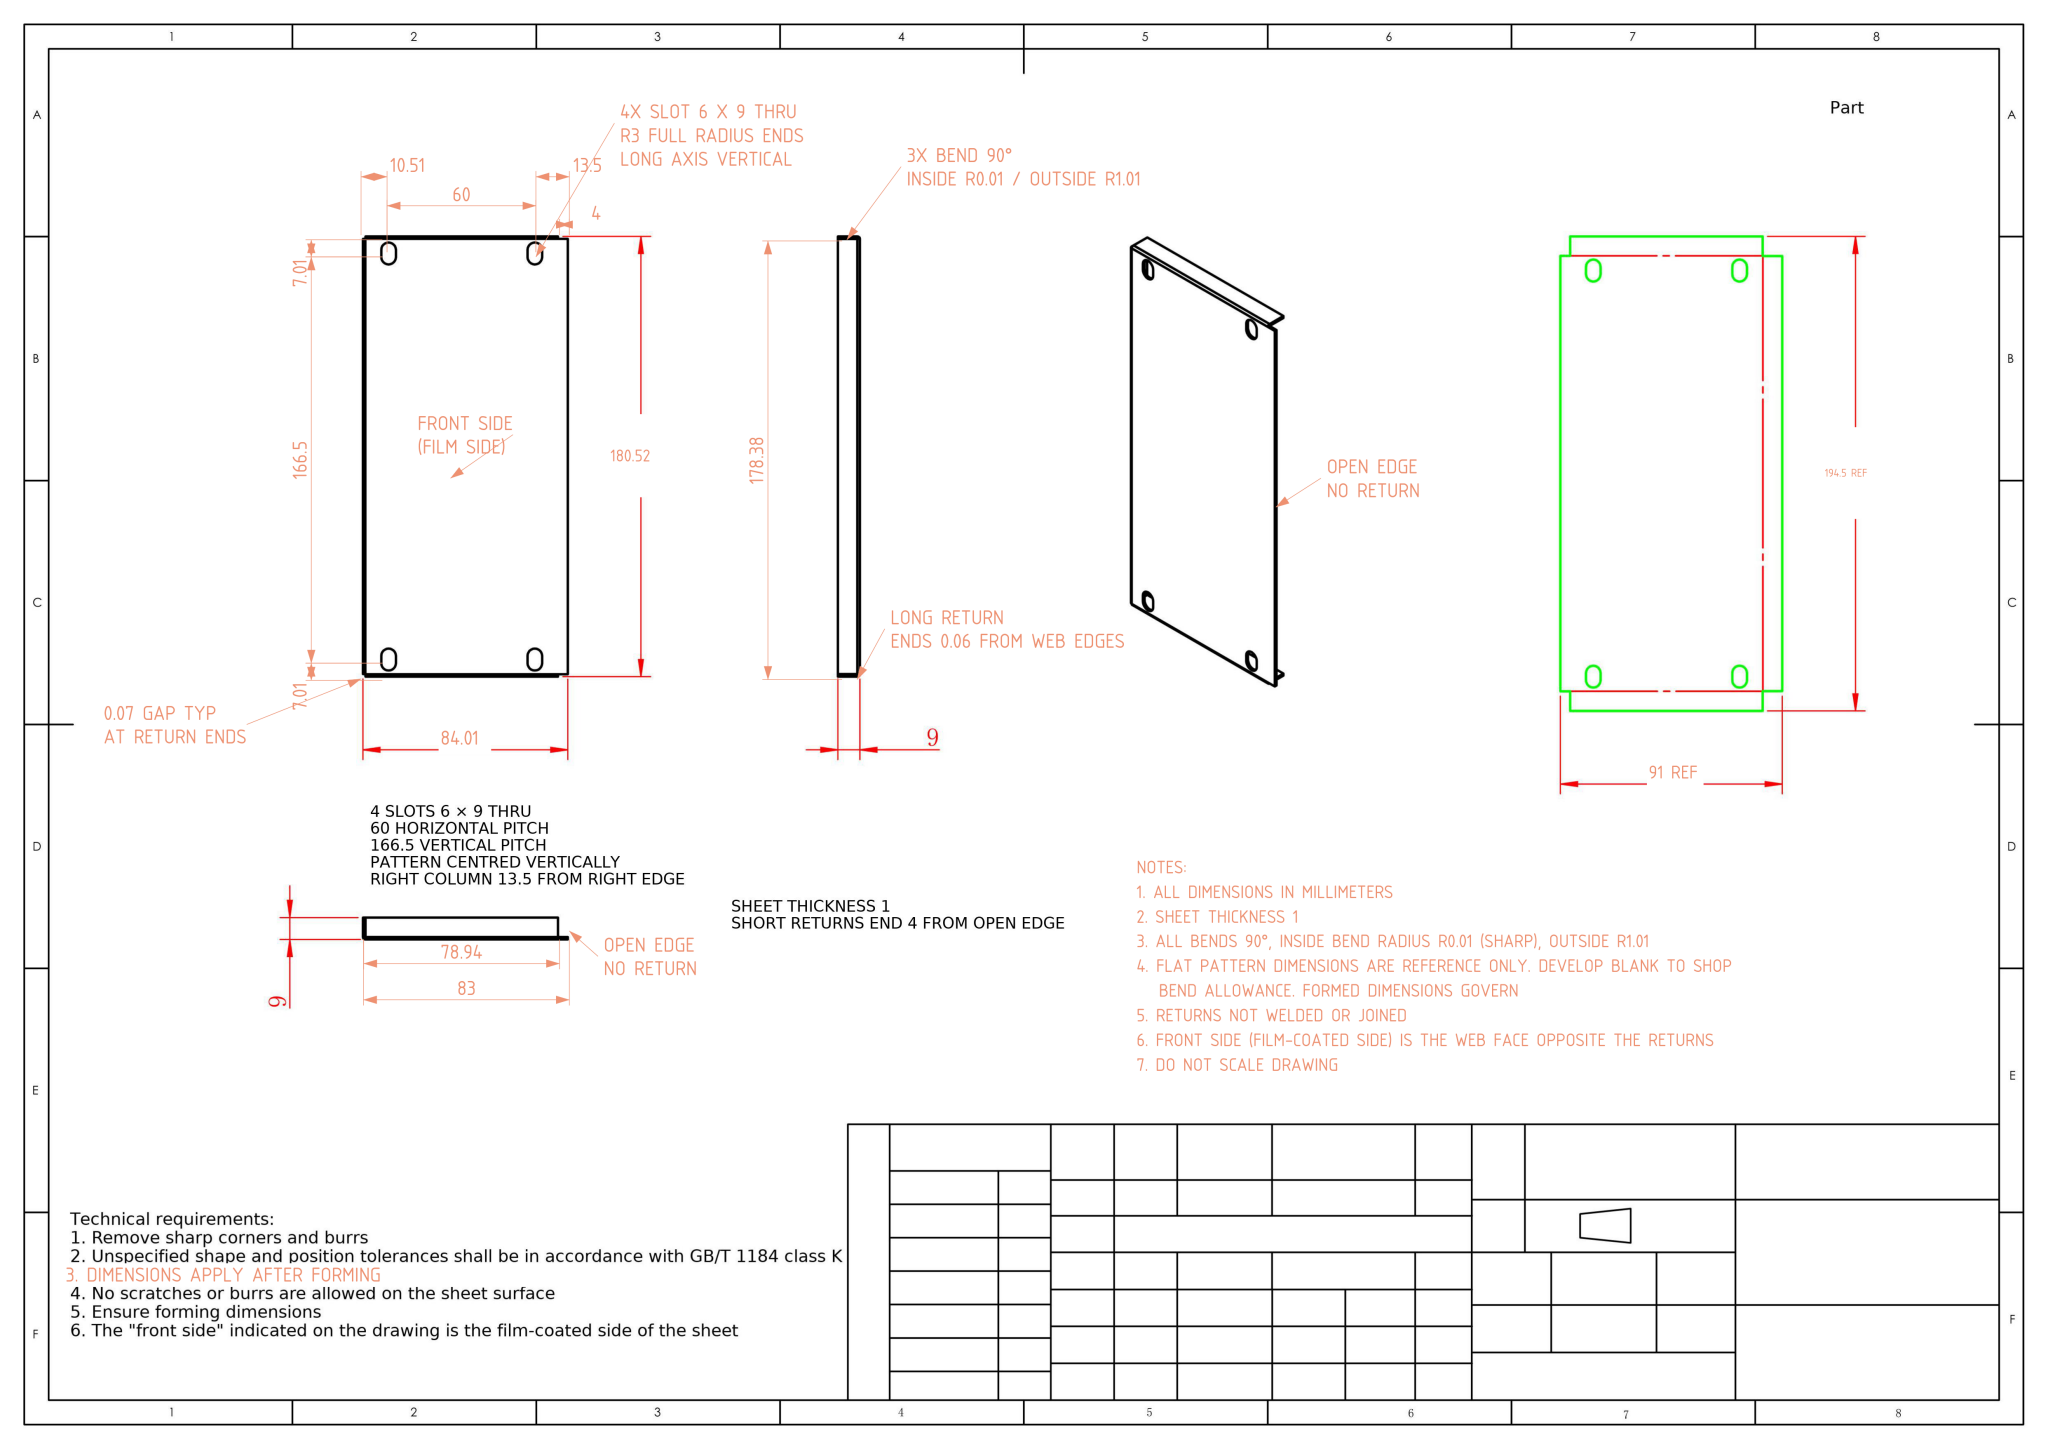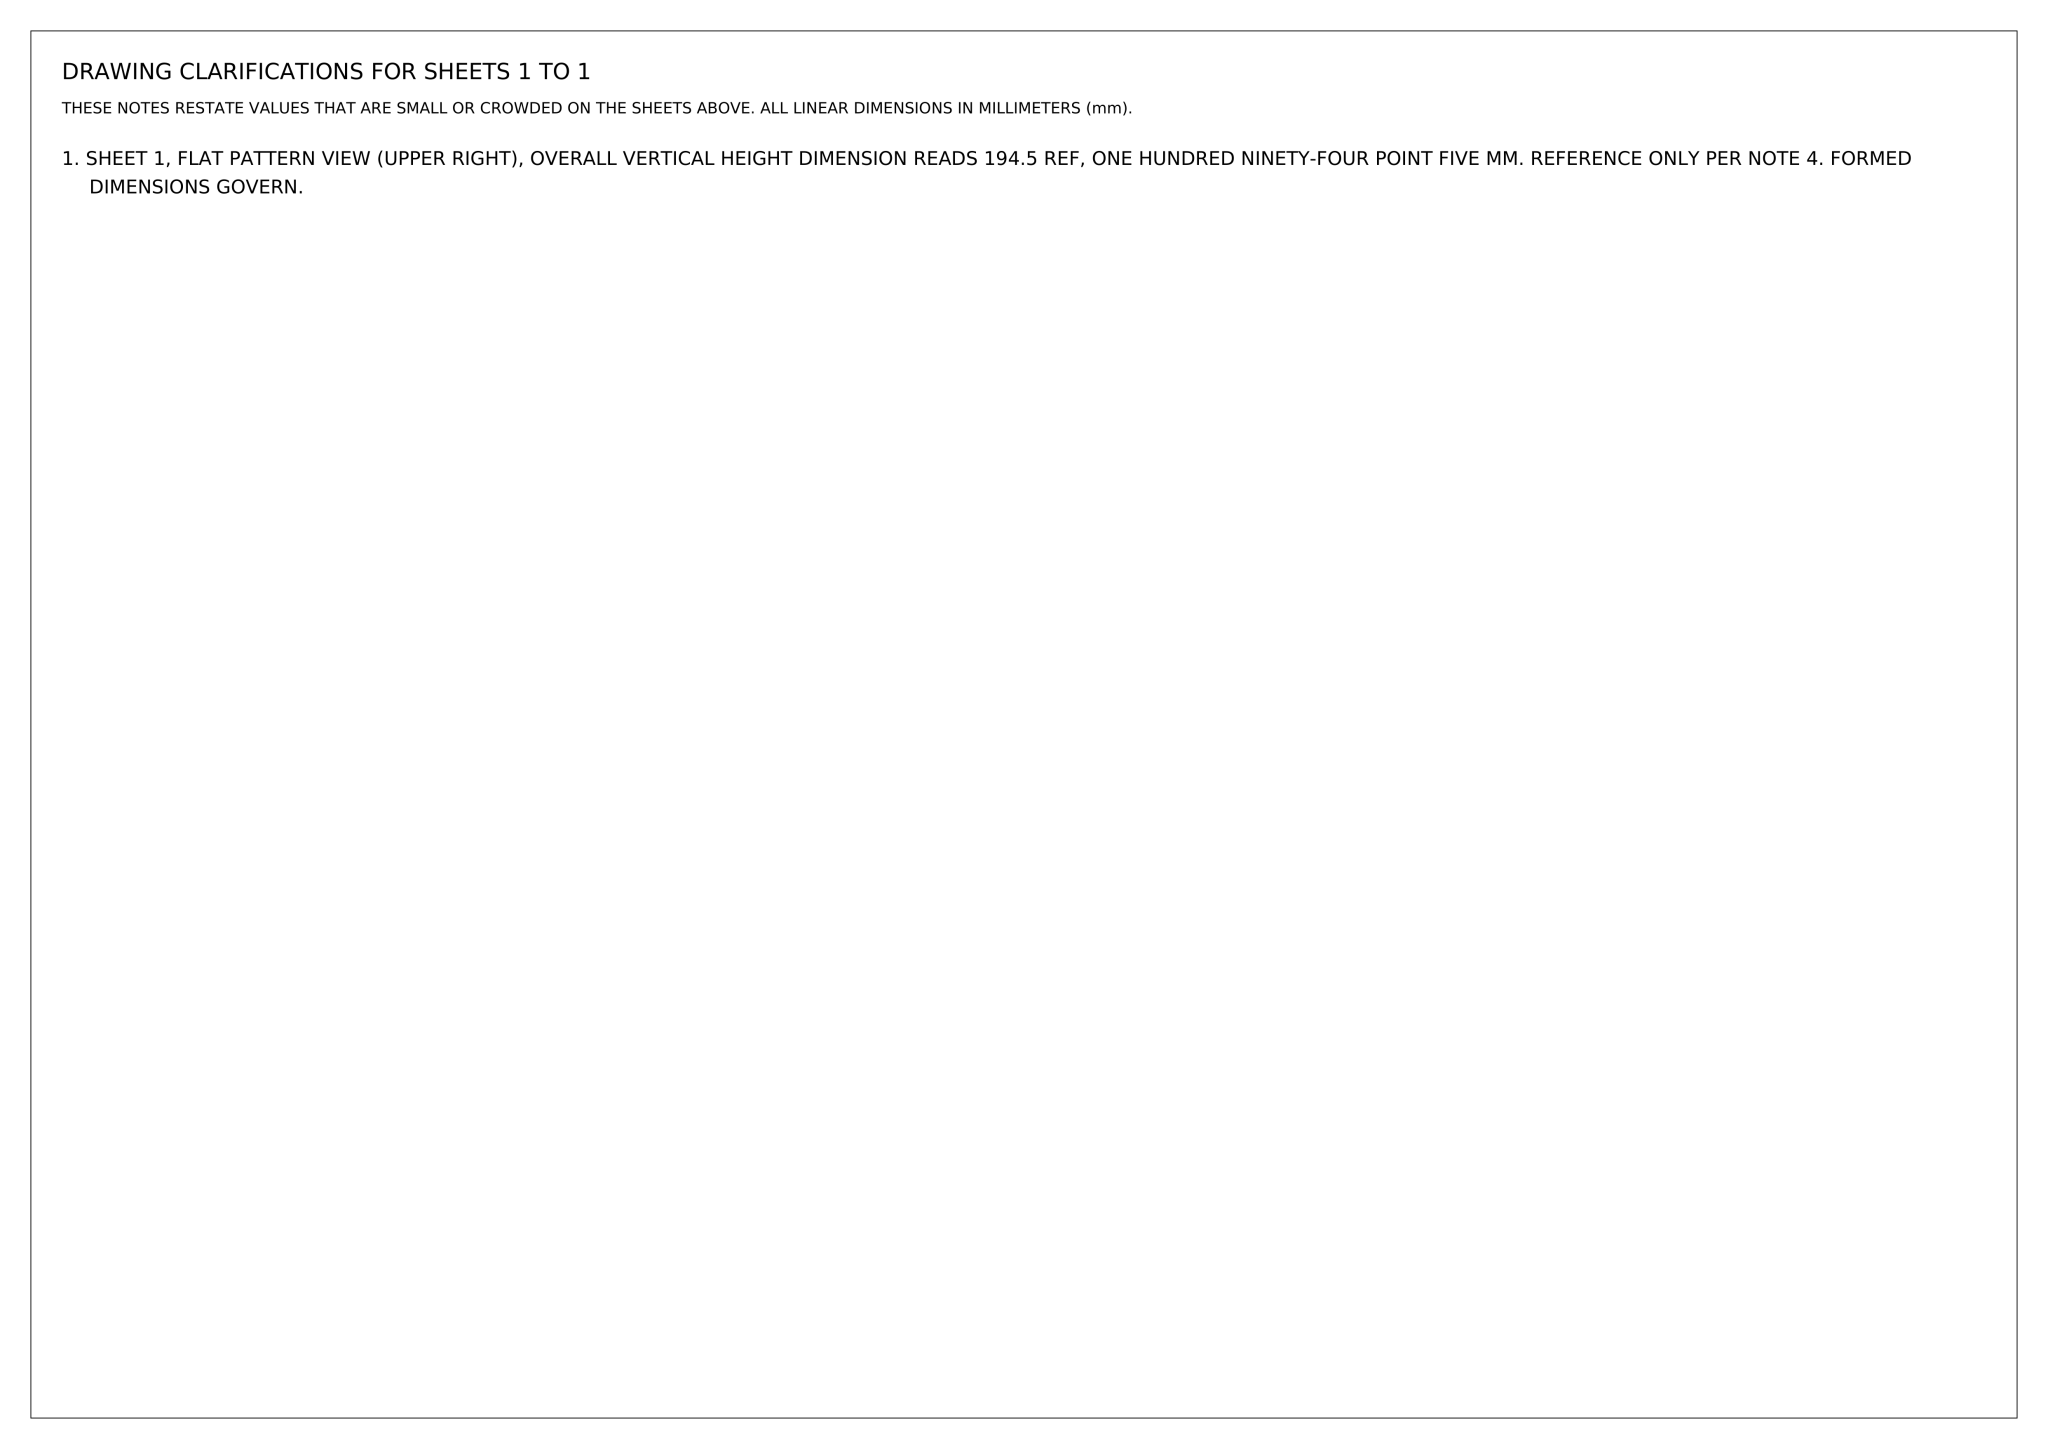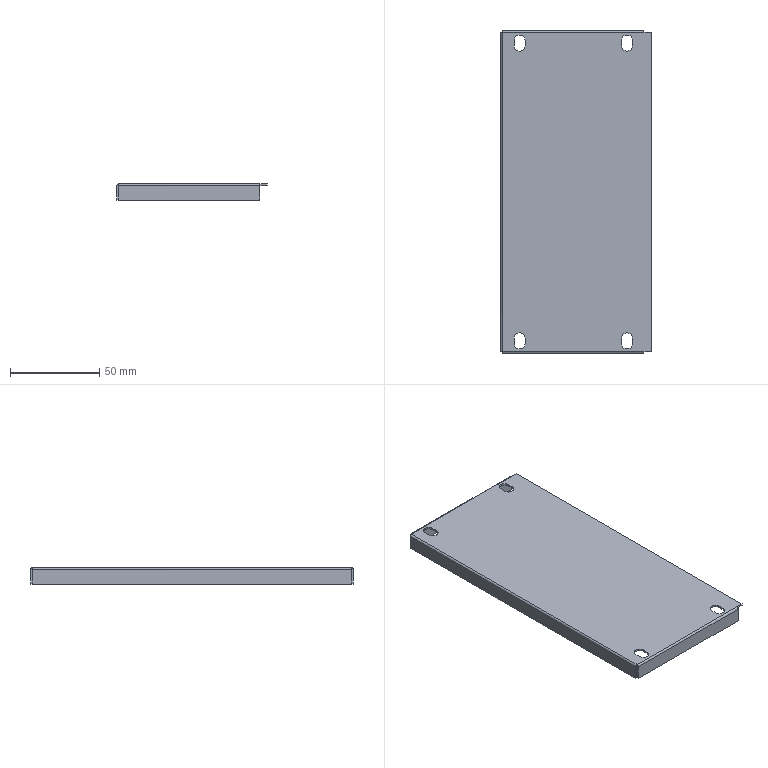Part | NX | mm | 1 solid | 48 faces | box 84.01 x 180.52 x 9 mm | volume 17587 mm3 | plane 30 | cylinder 14 | spline 4 | commonest cylinder face diameters 6 x8 2.02 x3 0.02 x3